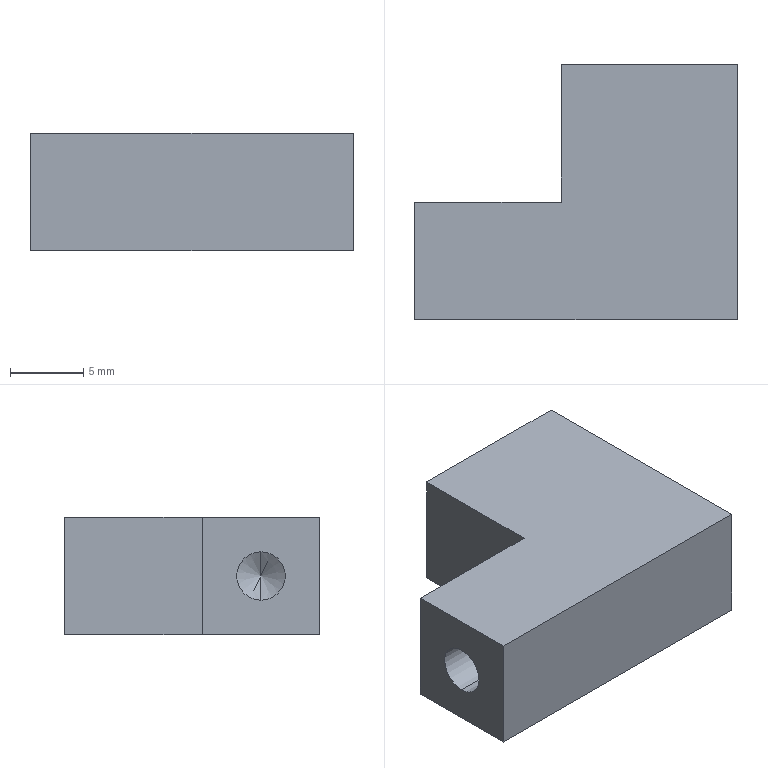Component | SolidWorks | 7.1.02.0001.00.00-0054-1 | 1 solid | 12 faces | box 22 x 17.4 x 8 mm | volume 2221 mm3 | plane 8 | cylinder 2 | cone 2 | commonest cylinder face diameters 3.3 x2
build123d program:
from build123d import *

# Parameters (mm, degrees)
BOSS_EXTRUDE1_DEPTH       = 8
M4X0_7_TAPPED_HOLE1_D     = 3.3
M4X0_7_TAPPED_HOLE1_DEPTH = 10.1
M4X0_7_TAPPED_HOLE1_TIP   = 0.9914


with BuildPart() as part:
    # Sketch1 → Boss-Extrude1 (new body)
    with BuildSketch(Plane.XY):
        Polygon((-11, 0.7), (-1, 0.7), (-1, -8.7), (11, -8.7), (11, 8.7), (-11, 8.7), align=None)
    extrude(amount=BOSS_EXTRUDE1_DEPTH)

    # M4x0.7 Tapped Hole1
    with Locations(Plane(origin=(-11, 4.7, 4), x_dir=(0, 0, -1), z_dir=(-1, 0, 0))):
        with Locations((0, 0)):
            Hole(M4X0_7_TAPPED_HOLE1_D / 2, depth=M4X0_7_TAPPED_HOLE1_DEPTH)
            with Locations((0, 0, -(M4X0_7_TAPPED_HOLE1_DEPTH + M4X0_7_TAPPED_HOLE1_TIP / 2))):  # 118° drill point
                Cone(0, M4X0_7_TAPPED_HOLE1_D / 2, M4X0_7_TAPPED_HOLE1_TIP, mode=Mode.SUBTRACT)


solid = part.part

# Placed as in the assembly
solid = solid.moved(Location((-36.964, 37.616, 22.5), (180, 0, 0)))
STEP:
#1=COLOUR_RGB('',0.7922,0.8196,0.9333);
#2=FILL_AREA_STYLE_COLOUR('',#1);
#3=FILL_AREA_STYLE('',(#2));
#4=SURFACE_STYLE_FILL_AREA(#3);
#5=SURFACE_SIDE_STYLE('',(#4));
#6=SURFACE_STYLE_USAGE(.BOTH.,#5);
#7=PRESENTATION_STYLE_ASSIGNMENT((#6));
#8=CARTESIAN_POINT('',(-1.491,1.296,0.7933));
#9=VERTEX_POINT('',#8);
#10=CARTESIAN_POINT('',(-1.491,1.296,0.6634));
#11=VERTEX_POINT('',#10);
#12=CARTESIAN_POINT('',(-1.491,1.296,0.7283));
#13=DIRECTION('',(-1.,-0.,0.));
#14=DIRECTION('',(0.,0.,-1.));
#15=AXIS2_PLACEMENT_3D('',#12,#13,#14);
#16=CIRCLE('',#15,0.06496);
#17=EDGE_CURVE('',#9,#11,#16,.T.);
#18=ORIENTED_EDGE('',*,*,#17,.F.);
#19=CARTESIAN_POINT('',(-1.888,1.296,0.7933));
#20=VERTEX_POINT('',#19);
#21=CARTESIAN_POINT('',(-1.888,1.296,0.7933));
#22=DIRECTION('',(-1.,-0.,0.));
#23=VECTOR('',#22,39.37);
#24=LINE('',#21,#23);
#25=EDGE_CURVE('',#9,#20,#24,.T.);
#26=ORIENTED_EDGE('',*,*,#25,.T.);
#27=CARTESIAN_POINT('',(-1.888,1.296,0.6634));
#28=VERTEX_POINT('',#27);
#29=CARTESIAN_POINT('',(-1.888,1.296,0.7283));
#30=DIRECTION('',(-1.,-0.,0.));
#31=DIRECTION('',(0.,0.,-1.));
#32=AXIS2_PLACEMENT_3D('',#29,#30,#31);
#33=CIRCLE('',#32,0.06496);
#34=EDGE_CURVE('',#20,#28,#33,.T.);
#35=ORIENTED_EDGE('',*,*,#34,.T.);
#36=CARTESIAN_POINT('',(-1.888,1.296,0.6634));
#37=DIRECTION('',(-1.,-0.,0.));
#38=VECTOR('',#37,39.37);
#39=LINE('',#36,#38);
#40=EDGE_CURVE('',#11,#28,#39,.T.);
#41=ORIENTED_EDGE('',*,*,#40,.F.);
#42=EDGE_LOOP('',(#18,#26,#35,#41));
#43=FACE_OUTER_BOUND('',#42,.T.);
#44=CARTESIAN_POINT('',(-1.888,1.296,0.7283));
#45=DIRECTION('',(-1.,-0.,0.));
#46=DIRECTION('',(0.,0.,-1.));
#47=AXIS2_PLACEMENT_3D('',#44,#45,#46);
#48=CYLINDRICAL_SURFACE('',#47,0.06496);
#49=ADVANCED_FACE('',(#43),#48,.F.);
#50=CARTESIAN_POINT('',(-1.452,1.296,0.7283));
#51=VERTEX_POINT('',#50);
#52=CARTESIAN_POINT('',(-1.491,1.296,0.6634));
#53=DIRECTION('',(-0.515,0.,-0.8572));
#54=VECTOR('',#53,39.37);
#55=LINE('',#52,#54);
#56=EDGE_CURVE('',#51,#11,#55,.T.);
#57=ORIENTED_EDGE('',*,*,#56,.F.);
#58=CARTESIAN_POINT('',(-1.491,1.296,0.7933));
#59=DIRECTION('',(-0.515,-0.,0.8572));
#60=VECTOR('',#59,39.37);
#61=LINE('',#58,#60);
#62=EDGE_CURVE('',#51,#9,#61,.T.);
#63=ORIENTED_EDGE('',*,*,#62,.T.);
#64=ORIENTED_EDGE('',*,*,#17,.T.);
#65=EDGE_LOOP('',(#57,#63,#64));
#66=FACE_OUTER_BOUND('',#65,.T.);
#67=CARTESIAN_POINT('',(-1.491,1.296,0.7283));
#68=DIRECTION('',(-1.,-0.,0.));
#69=DIRECTION('',(0.,0.,-1.));
#70=AXIS2_PLACEMENT_3D('',#67,#68,#69);
#71=CONICAL_SURFACE('',#70,0.06496,1.03);
#72=ADVANCED_FACE('',(#66),#71,.F.);
#73=CARTESIAN_POINT('',(-1.888,1.296,0.7283));
#74=DIRECTION('',(-1.,-0.,0.));
#75=DIRECTION('',(0.,0.,-1.));
#76=AXIS2_PLACEMENT_3D('',#73,#74,#75);
#77=CIRCLE('',#76,0.06496);
#78=EDGE_CURVE('',#28,#20,#77,.T.);
#79=ORIENTED_EDGE('',*,*,#78,.F.);
#80=ORIENTED_EDGE('',*,*,#34,.F.);
#81=EDGE_LOOP('',(#79,#80));
#82=FACE_BOUND('',#81,.T.);
#83=CARTESIAN_POINT('',(-1.888,1.138,0.8858));
#84=VERTEX_POINT('',#83);
#85=CARTESIAN_POINT('',(-1.888,1.453,0.8858));
#86=VERTEX_POINT('',#85);
#87=CARTESIAN_POINT('',(-1.888,1.138,0.8858));
#88=DIRECTION('',(0.,1.,0.));
#89=VECTOR('',#88,39.37);
#90=LINE('',#87,#89);
#91=EDGE_CURVE('',#84,#86,#90,.T.);
#92=ORIENTED_EDGE('',*,*,#91,.T.);
#93=CARTESIAN_POINT('',(-1.888,1.453,0.5709));
#94=VERTEX_POINT('',#93);
#95=CARTESIAN_POINT('',(-1.888,1.453,0.5709));
#96=DIRECTION('',(0.,-0.,1.));
#97=VECTOR('',#96,39.37);
#98=LINE('',#95,#97);
#99=EDGE_CURVE('',#94,#86,#98,.T.);
#100=ORIENTED_EDGE('',*,*,#99,.F.);
#101=CARTESIAN_POINT('',(-1.888,1.138,0.5709));
#102=VERTEX_POINT('',#101);
#103=CARTESIAN_POINT('',(-1.888,1.138,0.5709));
#104=DIRECTION('',(0.,1.,0.));
#105=VECTOR('',#104,39.37);
#106=LINE('',#103,#105);
#107=EDGE_CURVE('',#102,#94,#106,.T.);
#108=ORIENTED_EDGE('',*,*,#107,.F.);
#109=CARTESIAN_POINT('',(-1.888,1.138,0.5709));
#110=DIRECTION('',(0.,-0.,1.));
#111=VECTOR('',#110,39.37);
#112=LINE('',#109,#111);
#113=EDGE_CURVE('',#102,#84,#112,.T.);
#114=ORIENTED_EDGE('',*,*,#113,.T.);
#115=EDGE_LOOP('',(#92,#100,#108,#114));
#116=FACE_OUTER_BOUND('',#115,.T.);
#117=CARTESIAN_POINT('',(-1.888,1.138,0.5709));
#118=DIRECTION('',(1.,0.,-0.));
#119=DIRECTION('',(0.,-0.,1.));
#120=AXIS2_PLACEMENT_3D('',#117,#118,#119);
#121=PLANE('',#120);
#122=ADVANCED_FACE('',(#82,#116),#121,.F.);
#123=CARTESIAN_POINT('',(-1.495,1.453,0.8858));
#124=VERTEX_POINT('',#123);
#125=CARTESIAN_POINT('',(-1.888,1.453,0.8858));
#126=DIRECTION('',(1.,0.,-0.));
#127=VECTOR('',#126,39.37);
#128=LINE('',#125,#127);
#129=EDGE_CURVE('',#86,#124,#128,.T.);
#130=ORIENTED_EDGE('',*,*,#129,.T.);
#131=CARTESIAN_POINT('',(-1.495,1.453,0.5709));
#132=VERTEX_POINT('',#131);
#133=CARTESIAN_POINT('',(-1.495,1.453,0.5709));
#134=DIRECTION('',(0.,-0.,1.));
#135=VECTOR('',#134,39.37);
#136=LINE('',#133,#135);
#137=EDGE_CURVE('',#132,#124,#136,.T.);
#138=ORIENTED_EDGE('',*,*,#137,.F.);
#139=CARTESIAN_POINT('',(-1.888,1.453,0.5709));
#140=DIRECTION('',(1.,0.,-0.));
#141=VECTOR('',#140,39.37);
#142=LINE('',#139,#141);
#143=EDGE_CURVE('',#94,#132,#142,.T.);
#144=ORIENTED_EDGE('',*,*,#143,.F.);
#145=ORIENTED_EDGE('',*,*,#99,.T.);
#146=EDGE_LOOP('',(#130,#138,#144,#145));
#147=FACE_OUTER_BOUND('',#146,.T.);
#148=CARTESIAN_POINT('',(-1.888,1.453,0.5709));
#149=DIRECTION('',(-0.,-1.,-0.));
#150=DIRECTION('',(-0.,0.,-1.));
#151=AXIS2_PLACEMENT_3D('',#148,#149,#150);
#152=PLANE('',#151);
#153=ADVANCED_FACE('',(#147),#152,.F.);
#154=CARTESIAN_POINT('',(-1.495,1.823,0.8858));
#155=VERTEX_POINT('',#154);
#156=CARTESIAN_POINT('',(-1.495,1.453,0.8858));
#157=DIRECTION('',(0.,1.,0.));
#158=VECTOR('',#157,39.37);
#159=LINE('',#156,#158);
#160=EDGE_CURVE('',#124,#155,#159,.T.);
#161=ORIENTED_EDGE('',*,*,#160,.T.);
#162=CARTESIAN_POINT('',(-1.495,1.823,0.5709));
#163=VERTEX_POINT('',#162);
#164=CARTESIAN_POINT('',(-1.495,1.823,0.5709));
#165=DIRECTION('',(0.,-0.,1.));
#166=VECTOR('',#165,39.37);
#167=LINE('',#164,#166);
#168=EDGE_CURVE('',#163,#155,#167,.T.);
#169=ORIENTED_EDGE('',*,*,#168,.F.);
#170=CARTESIAN_POINT('',(-1.495,1.453,0.5709));
#171=DIRECTION('',(0.,1.,0.));
#172=VECTOR('',#171,39.37);
#173=LINE('',#170,#172);
#174=EDGE_CURVE('',#132,#163,#173,.T.);
#175=ORIENTED_EDGE('',*,*,#174,.F.);
#176=ORIENTED_EDGE('',*,*,#137,.T.);
#177=EDGE_LOOP('',(#161,#169,#175,#176));
#178=FACE_OUTER_BOUND('',#177,.T.);
#179=CARTESIAN_POINT('',(-1.495,1.453,0.5709));
#180=DIRECTION('',(1.,-0.,-0.));
#181=DIRECTION('',(-0.,-1.,-0.));
#182=AXIS2_PLACEMENT_3D('',#179,#180,#181);
#183=PLANE('',#182);
#184=ADVANCED_FACE('',(#178),#183,.F.);
#185=CARTESIAN_POINT('',(-1.022,1.823,0.8858));
#186=VERTEX_POINT('',#185);
#187=CARTESIAN_POINT('',(-1.495,1.823,0.8858));
#188=DIRECTION('',(1.,0.,-0.));
#189=VECTOR('',#188,39.37);
#190=LINE('',#187,#189);
#191=EDGE_CURVE('',#155,#186,#190,.T.);
#192=ORIENTED_EDGE('',*,*,#191,.T.);
#193=CARTESIAN_POINT('',(-1.022,1.823,0.5709));
#194=VERTEX_POINT('',#193);
#195=CARTESIAN_POINT('',(-1.022,1.823,0.5709));
#196=DIRECTION('',(0.,-0.,1.));
#197=VECTOR('',#196,39.37);
#198=LINE('',#195,#197);
#199=EDGE_CURVE('',#194,#186,#198,.T.);
#200=ORIENTED_EDGE('',*,*,#199,.F.);
#201=CARTESIAN_POINT('',(-1.495,1.823,0.5709));
#202=DIRECTION('',(1.,0.,-0.));
#203=VECTOR('',#202,39.37);
#204=LINE('',#201,#203);
#205=EDGE_CURVE('',#163,#194,#204,.T.);
#206=ORIENTED_EDGE('',*,*,#205,.F.);
#207=ORIENTED_EDGE('',*,*,#168,.T.);
#208=EDGE_LOOP('',(#192,#200,#206,#207));
#209=FACE_OUTER_BOUND('',#208,.T.);
#210=CARTESIAN_POINT('',(-1.495,1.823,0.5709));
#211=DIRECTION('',(-0.,-1.,-0.));
#212=DIRECTION('',(-0.,0.,-1.));
#213=AXIS2_PLACEMENT_3D('',#210,#211,#212);
#214=PLANE('',#213);
#215=ADVANCED_FACE('',(#209),#214,.F.);
#216=CARTESIAN_POINT('',(-1.022,1.138,0.8858));
#217=VERTEX_POINT('',#216);
#218=CARTESIAN_POINT('',(-1.022,1.138,0.8858));
#219=DIRECTION('',(-0.,-1.,-0.));
#220=VECTOR('',#219,39.37);
#221=LINE('',#218,#220);
#222=EDGE_CURVE('',#186,#217,#221,.T.);
#223=ORIENTED_EDGE('',*,*,#222,.T.);
#224=CARTESIAN_POINT('',(-1.022,1.138,0.5709));
#225=VERTEX_POINT('',#224);
#226=CARTESIAN_POINT('',(-1.022,1.138,0.5709));
#227=DIRECTION('',(0.,-0.,1.));
#228=VECTOR('',#227,39.37);
#229=LINE('',#226,#228);
#230=EDGE_CURVE('',#225,#217,#229,.T.);
#231=ORIENTED_EDGE('',*,*,#230,.F.);
#232=CARTESIAN_POINT('',(-1.022,1.138,0.5709));
#233=DIRECTION('',(-0.,-1.,-0.));
#234=VECTOR('',#233,39.37);
#235=LINE('',#232,#234);
#236=EDGE_CURVE('',#194,#225,#235,.T.);
#237=ORIENTED_EDGE('',*,*,#236,.F.);
#238=ORIENTED_EDGE('',*,*,#199,.T.);
#239=EDGE_LOOP('',(#223,#231,#237,#238));
#240=FACE_OUTER_BOUND('',#239,.T.);
#241=CARTESIAN_POINT('',(-1.022,1.138,0.5709));
#242=DIRECTION('',(-1.,-0.,0.));
#243=DIRECTION('',(-0.,0.,-1.));
#244=AXIS2_PLACEMENT_3D('',#241,#242,#243);
#245=PLANE('',#244);
#246=ADVANCED_FACE('',(#240),#245,.F.);
#247=CARTESIAN_POINT('',(-1.888,1.138,0.8858));
#248=DIRECTION('',(-1.,-0.,0.));
#249=VECTOR('',#248,39.37);
#250=LINE('',#247,#249);
#251=EDGE_CURVE('',#217,#84,#250,.T.);
#252=ORIENTED_EDGE('',*,*,#251,.T.);
#253=ORIENTED_EDGE('',*,*,#113,.F.);
#254=CARTESIAN_POINT('',(-1.888,1.138,0.5709));
#255=DIRECTION('',(-1.,-0.,0.));
#256=VECTOR('',#255,39.37);
#257=LINE('',#254,#256);
#258=EDGE_CURVE('',#225,#102,#257,.T.);
#259=ORIENTED_EDGE('',*,*,#258,.F.);
#260=ORIENTED_EDGE('',*,*,#230,.T.);
#261=EDGE_LOOP('',(#252,#253,#259,#260));
#262=FACE_OUTER_BOUND('',#261,.T.);
#263=CARTESIAN_POINT('',(-1.888,1.138,0.5709));
#264=DIRECTION('',(0.,1.,0.));
#265=DIRECTION('',(0.,-0.,1.));
#266=AXIS2_PLACEMENT_3D('',#263,#264,#265);
#267=PLANE('',#266);
#268=ADVANCED_FACE('',(#262),#267,.F.);
#269=ORIENTED_EDGE('',*,*,#107,.T.);
#270=ORIENTED_EDGE('',*,*,#143,.T.);
#271=ORIENTED_EDGE('',*,*,#174,.T.);
#272=ORIENTED_EDGE('',*,*,#205,.T.);
#273=ORIENTED_EDGE('',*,*,#236,.T.);
#274=ORIENTED_EDGE('',*,*,#258,.T.);
#275=EDGE_LOOP('',(#269,#270,#271,#272,#273,#274));
#276=FACE_OUTER_BOUND('',#275,.T.);
#277=CARTESIAN_POINT('',(-1.455,1.481,0.5709));
#278=DIRECTION('',(-0.,0.,-1.));
#279=DIRECTION('',(1.,0.,-0.));
#280=AXIS2_PLACEMENT_3D('',#277,#278,#279);
#281=PLANE('',#280);
#282=ADVANCED_FACE('',(#276),#281,.T.);
#283=ORIENTED_EDGE('',*,*,#91,.F.);
#284=ORIENTED_EDGE('',*,*,#251,.F.);
#285=ORIENTED_EDGE('',*,*,#222,.F.);
#286=ORIENTED_EDGE('',*,*,#191,.F.);
#287=ORIENTED_EDGE('',*,*,#160,.F.);
#288=ORIENTED_EDGE('',*,*,#129,.F.);
#289=EDGE_LOOP('',(#283,#284,#285,#286,#287,#288));
#290=FACE_OUTER_BOUND('',#289,.T.);
#291=CARTESIAN_POINT('',(-1.455,1.481,0.8858));
#292=DIRECTION('',(-0.,0.,-1.));
#293=DIRECTION('',(1.,0.,-0.));
#294=AXIS2_PLACEMENT_3D('',#291,#292,#293);
#295=PLANE('',#294);
#296=ADVANCED_FACE('',(#290),#295,.F.);
#297=ORIENTED_EDGE('',*,*,#62,.F.);
#298=ORIENTED_EDGE('',*,*,#56,.T.);
#299=CARTESIAN_POINT('',(-1.491,1.296,0.7283));
#300=DIRECTION('',(-1.,-0.,0.));
#301=DIRECTION('',(0.,0.,-1.));
#302=AXIS2_PLACEMENT_3D('',#299,#300,#301);
#303=CIRCLE('',#302,0.06496);
#304=EDGE_CURVE('',#11,#9,#303,.T.);
#305=ORIENTED_EDGE('',*,*,#304,.T.);
#306=EDGE_LOOP('',(#297,#298,#305));
#307=FACE_OUTER_BOUND('',#306,.T.);
#308=CARTESIAN_POINT('',(-1.491,1.296,0.7283));
#309=DIRECTION('',(-1.,-0.,0.));
#310=DIRECTION('',(0.,0.,-1.));
#311=AXIS2_PLACEMENT_3D('',#308,#309,#310);
#312=CONICAL_SURFACE('',#311,0.06496,1.03);
#313=ADVANCED_FACE('',(#307),#312,.F.);
#314=ORIENTED_EDGE('',*,*,#25,.F.);
#315=ORIENTED_EDGE('',*,*,#304,.F.);
#316=ORIENTED_EDGE('',*,*,#40,.T.);
#317=ORIENTED_EDGE('',*,*,#78,.T.);
#318=EDGE_LOOP('',(#314,#315,#316,#317));
#319=FACE_OUTER_BOUND('',#318,.T.);
#320=CARTESIAN_POINT('',(-1.888,1.296,0.7283));
#321=DIRECTION('',(-1.,-0.,0.));
#322=DIRECTION('',(0.,0.,-1.));
#323=AXIS2_PLACEMENT_3D('',#320,#321,#322);
#324=CYLINDRICAL_SURFACE('',#323,0.06496);
#325=ADVANCED_FACE('',(#319),#324,.F.);
#326=CLOSED_SHELL('',(#49,#72,#122,#153,#184,#215,#246,#268,#282,#296,#313,#325));
#327=MANIFOLD_SOLID_BREP('',#326);
#328=STYLED_ITEM('',(#7),#327);
#329=(LENGTH_UNIT()NAMED_UNIT(*)SI_UNIT($,.METRE.));
#330=LENGTH_MEASURE_WITH_UNIT(LENGTH_MEASURE(0.0254),#329);
#331=DIMENSIONAL_EXPONENTS(1.,0.,0.,0.,0.,0.,0.);
#332=(CONVERSION_BASED_UNIT('',#330)LENGTH_UNIT()NAMED_UNIT(#331));
#333=UNCERTAINTY_MEASURE_WITH_UNIT(LENGTH_MEASURE(0.00001),#332,'','');
#334=(NAMED_UNIT(*)PLANE_ANGLE_UNIT()SI_UNIT($,.RADIAN.));
#335=(NAMED_UNIT(*)SI_UNIT($,.STERADIAN.)SOLID_ANGLE_UNIT());
#336=(GEOMETRIC_REPRESENTATION_CONTEXT(3)GLOBAL_UNCERTAINTY_ASSIGNED_CONTEXT((#333))GLOBAL_UNIT_ASSIGNED_CONTEXT((#332,#334,#335))REPRESENTATION_CONTEXT('',''));
#337=MECHANICAL_DESIGN_GEOMETRIC_PRESENTATION_REPRESENTATION('',(#328),#336);
#338=PRESENTATION_LAYER_ASSIGNMENT('','',(#328));
#339=CARTESIAN_POINT('',(0.,0.,0.));
#340=DIRECTION('',(0.,0.,1.));
#341=DIRECTION('',(1.,0.,0.));
#342=AXIS2_PLACEMENT_3D('',#339,#340,#341);
#343=(LENGTH_UNIT()NAMED_UNIT(*)SI_UNIT($,.METRE.));
#344=LENGTH_MEASURE_WITH_UNIT(LENGTH_MEASURE(0.0254),#343);
#345=DIMENSIONAL_EXPONENTS(1.,0.,0.,0.,0.,0.,0.);
#346=(CONVERSION_BASED_UNIT('',#344)LENGTH_UNIT()NAMED_UNIT(#345));
#347=UNCERTAINTY_MEASURE_WITH_UNIT(LENGTH_MEASURE(0.00001),#346,'','');
#348=(NAMED_UNIT(*)PLANE_ANGLE_UNIT()SI_UNIT($,.RADIAN.));
#349=(NAMED_UNIT(*)SI_UNIT($,.STERADIAN.)SOLID_ANGLE_UNIT());
#350=(GEOMETRIC_REPRESENTATION_CONTEXT(3)GLOBAL_UNCERTAINTY_ASSIGNED_CONTEXT((#347))GLOBAL_UNIT_ASSIGNED_CONTEXT((#346,#348,#349))REPRESENTATION_CONTEXT('',''));
#351=ADVANCED_BREP_SHAPE_REPRESENTATION('',(#327,#342),#350);